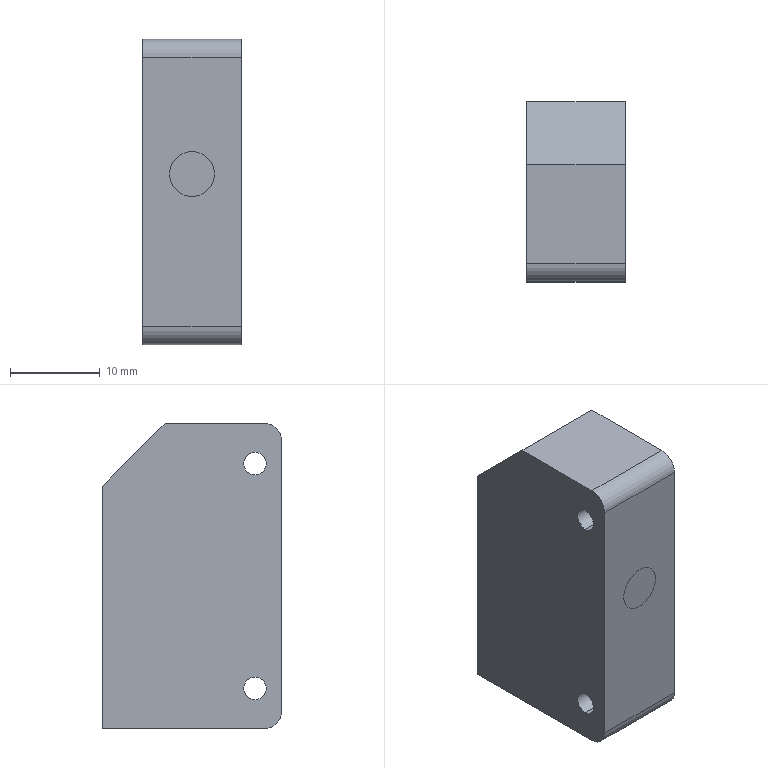Component | SolidWorks | MaterialDetectionSensor-1 | 1 solid | 14 faces | box 11 x 20 x 34 mm | volume 7084 mm3 | plane 8 | cylinder 6 | commonest cylinder face diameters 2.5 x4 4 x2
build123d program:
from build123d import *

# Parameters (mm, degrees)
SKETCH1_W           = 34
SKETCH1_H           = 20
BOSS_EXTRUDE1_DEPTH = 5.5
CUT_EXTRUDE1_DEPTH  = 23.583
M3_TAPPED_HOLE1_D   = 2.5
FILLET1_R           = 2


with BuildPart() as part:
    # Sketch1 → Boss-Extrude1 (new, symmetric)
    with BuildSketch(Plane.XY):
        Rectangle(SKETCH1_W, SKETCH1_H)
    extrude(amount=BOSS_EXTRUDE1_DEPTH, both=True)

    # Sketch2 → Cut-Extrude1 (cut, through all)
    with BuildSketch(Plane.XY.offset(5.5)):
        Polygon((-17, 10), (-10, 10), (-17, 3), align=None)
    extrude(amount=-CUT_EXTRUDE1_DEPTH, mode=Mode.SUBTRACT)

    # M3 Tapped Hole1 (through all)
    with Locations(Plane.XY.offset(5.5)):
        with Locations((-12.5, -7), (12.5, -7)):
            Hole(M3_TAPPED_HOLE1_D / 2)

    # Fillet1
    fillet1_edges = [part.edges().sort_by_distance(p)[0] for p in [
        (17, -10, 0),
        (-17, -10, 0),
    ]]
    fillet(fillet1_edges, radius=FILLET1_R)


solid = part.part

# Placed as in the assembly
solid = solid.moved(Location((-217.5, 1265.5, 90), (0, 90, 0)))
STEP:
#1=CARTESIAN_POINT('',(-8.78,49.547,4.085));
#2=VERTEX_POINT('',#1);
#3=CARTESIAN_POINT('',(-8.78,49.547,3.986));
#4=VERTEX_POINT('',#3);
#5=CARTESIAN_POINT('',(-8.78,49.547,4.035));
#6=DIRECTION('',(1.,0.,0.));
#7=DIRECTION('',(0.,0.,-1.));
#8=AXIS2_PLACEMENT_3D('',#5,#6,#7);
#9=CIRCLE('',#8,0.04921);
#10=EDGE_CURVE('',#2,#4,#9,.T.);
#11=ORIENTED_EDGE('',*,*,#10,.F.);
#12=CARTESIAN_POINT('',(-8.346,49.547,4.085));
#13=VERTEX_POINT('',#12);
#14=CARTESIAN_POINT('',(-8.346,49.547,4.085));
#15=DIRECTION('',(1.,0.,0.));
#16=VECTOR('',#15,39.37);
#17=LINE('',#14,#16);
#18=EDGE_CURVE('',#2,#13,#17,.T.);
#19=ORIENTED_EDGE('',*,*,#18,.T.);
#20=CARTESIAN_POINT('',(-8.346,49.547,3.986));
#21=VERTEX_POINT('',#20);
#22=CARTESIAN_POINT('',(-8.346,49.547,4.035));
#23=DIRECTION('',(1.,0.,0.));
#24=DIRECTION('',(0.,0.,-1.));
#25=AXIS2_PLACEMENT_3D('',#22,#23,#24);
#26=CIRCLE('',#25,0.04921);
#27=EDGE_CURVE('',#13,#21,#26,.T.);
#28=ORIENTED_EDGE('',*,*,#27,.T.);
#29=CARTESIAN_POINT('',(-8.346,49.547,3.986));
#30=DIRECTION('',(1.,0.,0.));
#31=VECTOR('',#30,39.37);
#32=LINE('',#29,#31);
#33=EDGE_CURVE('',#4,#21,#32,.T.);
#34=ORIENTED_EDGE('',*,*,#33,.F.);
#35=EDGE_LOOP('',(#11,#19,#28,#34));
#36=FACE_OUTER_BOUND('',#35,.T.);
#37=CARTESIAN_POINT('',(-8.346,49.547,4.035));
#38=DIRECTION('',(1.,0.,0.));
#39=DIRECTION('',(0.,0.,-1.));
#40=AXIS2_PLACEMENT_3D('',#37,#38,#39);
#41=CYLINDRICAL_SURFACE('',#40,0.04921);
#42=ADVANCED_FACE('',(#36),#41,.F.);
#43=CARTESIAN_POINT('',(-8.78,49.547,3.1));
#44=VERTEX_POINT('',#43);
#45=CARTESIAN_POINT('',(-8.78,49.547,3.002));
#46=VERTEX_POINT('',#45);
#47=CARTESIAN_POINT('',(-8.78,49.547,3.051));
#48=DIRECTION('',(1.,0.,0.));
#49=DIRECTION('',(0.,0.,-1.));
#50=AXIS2_PLACEMENT_3D('',#47,#48,#49);
#51=CIRCLE('',#50,0.04921);
#52=EDGE_CURVE('',#44,#46,#51,.T.);
#53=ORIENTED_EDGE('',*,*,#52,.F.);
#54=CARTESIAN_POINT('',(-8.346,49.547,3.1));
#55=VERTEX_POINT('',#54);
#56=CARTESIAN_POINT('',(-8.346,49.547,3.1));
#57=DIRECTION('',(1.,0.,0.));
#58=VECTOR('',#57,39.37);
#59=LINE('',#56,#58);
#60=EDGE_CURVE('',#44,#55,#59,.T.);
#61=ORIENTED_EDGE('',*,*,#60,.T.);
#62=CARTESIAN_POINT('',(-8.346,49.547,3.002));
#63=VERTEX_POINT('',#62);
#64=CARTESIAN_POINT('',(-8.346,49.547,3.051));
#65=DIRECTION('',(1.,0.,0.));
#66=DIRECTION('',(0.,0.,-1.));
#67=AXIS2_PLACEMENT_3D('',#64,#65,#66);
#68=CIRCLE('',#67,0.04921);
#69=EDGE_CURVE('',#55,#63,#68,.T.);
#70=ORIENTED_EDGE('',*,*,#69,.T.);
#71=CARTESIAN_POINT('',(-8.346,49.547,3.002));
#72=DIRECTION('',(1.,0.,0.));
#73=VECTOR('',#72,39.37);
#74=LINE('',#71,#73);
#75=EDGE_CURVE('',#46,#63,#74,.T.);
#76=ORIENTED_EDGE('',*,*,#75,.F.);
#77=EDGE_LOOP('',(#53,#61,#70,#76));
#78=FACE_OUTER_BOUND('',#77,.T.);
#79=CARTESIAN_POINT('',(-8.346,49.547,3.051));
#80=DIRECTION('',(1.,0.,0.));
#81=DIRECTION('',(0.,0.,-1.));
#82=AXIS2_PLACEMENT_3D('',#79,#80,#81);
#83=CYLINDRICAL_SURFACE('',#82,0.04921);
#84=ADVANCED_FACE('',(#78),#83,.F.);
#85=CARTESIAN_POINT('',(-8.346,49.429,4.134));
#86=VERTEX_POINT('',#85);
#87=CARTESIAN_POINT('',(-8.346,49.429,2.953));
#88=VERTEX_POINT('',#87);
#89=CARTESIAN_POINT('',(-8.346,49.429,4.213));
#90=DIRECTION('',(0.,-0.,-1.));
#91=VECTOR('',#90,39.37);
#92=LINE('',#89,#91);
#93=EDGE_CURVE('',#86,#88,#92,.T.);
#94=ORIENTED_EDGE('',*,*,#93,.F.);
#95=CARTESIAN_POINT('',(-8.78,49.429,4.134));
#96=VERTEX_POINT('',#95);
#97=CARTESIAN_POINT('',(-8.346,49.429,4.134));
#98=DIRECTION('',(-1.,-0.,0.));
#99=VECTOR('',#98,39.37);
#100=LINE('',#97,#99);
#101=EDGE_CURVE('',#86,#96,#100,.T.);
#102=ORIENTED_EDGE('',*,*,#101,.T.);
#103=CARTESIAN_POINT('',(-8.78,49.429,2.953));
#104=VERTEX_POINT('',#103);
#105=CARTESIAN_POINT('',(-8.78,49.429,4.213));
#106=DIRECTION('',(0.,-0.,-1.));
#107=VECTOR('',#106,39.37);
#108=LINE('',#105,#107);
#109=EDGE_CURVE('',#96,#104,#108,.T.);
#110=ORIENTED_EDGE('',*,*,#109,.T.);
#111=CARTESIAN_POINT('',(-8.346,49.429,2.953));
#112=DIRECTION('',(1.,0.,0.));
#113=VECTOR('',#112,39.37);
#114=LINE('',#111,#113);
#115=EDGE_CURVE('',#104,#88,#114,.T.);
#116=ORIENTED_EDGE('',*,*,#115,.T.);
#117=EDGE_LOOP('',(#94,#102,#110,#116));
#118=FACE_OUTER_BOUND('',#117,.T.);
#119=CARTESIAN_POINT('',(-8.465,49.429,3.622));
#120=VERTEX_POINT('',#119);
#121=CARTESIAN_POINT('',(-8.661,49.429,3.622));
#122=VERTEX_POINT('',#121);
#123=CARTESIAN_POINT('',(-8.563,49.429,3.622));
#124=DIRECTION('',(0.,-1.,0.));
#125=DIRECTION('',(1.,0.,0.));
#126=AXIS2_PLACEMENT_3D('',#123,#124,#125);
#127=CIRCLE('',#126,0.09843);
#128=EDGE_CURVE('',#120,#122,#127,.T.);
#129=ORIENTED_EDGE('',*,*,#128,.F.);
#130=CARTESIAN_POINT('',(-8.563,49.429,3.622));
#131=DIRECTION('',(0.,-1.,0.));
#132=DIRECTION('',(1.,0.,0.));
#133=AXIS2_PLACEMENT_3D('',#130,#131,#132);
#134=CIRCLE('',#133,0.09843);
#135=EDGE_CURVE('',#122,#120,#134,.T.);
#136=ORIENTED_EDGE('',*,*,#135,.F.);
#137=EDGE_LOOP('',(#129,#136));
#138=FACE_BOUND('',#137,.T.);
#139=CARTESIAN_POINT('',(-8.346,49.429,4.213));
#140=DIRECTION('',(-0.,1.,-0.));
#141=DIRECTION('',(1.,0.,0.));
#142=AXIS2_PLACEMENT_3D('',#139,#140,#141);
#143=PLANE('',#142);
#144=ADVANCED_FACE('',(#118,#138),#143,.F.);
#145=CARTESIAN_POINT('',(-8.346,49.508,2.874));
#146=VERTEX_POINT('',#145);
#147=CARTESIAN_POINT('',(-8.346,50.217,2.874));
#148=VERTEX_POINT('',#147);
#149=CARTESIAN_POINT('',(-8.346,50.217,2.874));
#150=DIRECTION('',(-0.,1.,-0.));
#151=VECTOR('',#150,39.37);
#152=LINE('',#149,#151);
#153=EDGE_CURVE('',#146,#148,#152,.T.);
#154=ORIENTED_EDGE('',*,*,#153,.F.);
#155=CARTESIAN_POINT('',(-8.78,49.508,2.874));
#156=VERTEX_POINT('',#155);
#157=CARTESIAN_POINT('',(-8.346,49.508,2.874));
#158=DIRECTION('',(-1.,-0.,0.));
#159=VECTOR('',#158,39.37);
#160=LINE('',#157,#159);
#161=EDGE_CURVE('',#146,#156,#160,.T.);
#162=ORIENTED_EDGE('',*,*,#161,.T.);
#163=CARTESIAN_POINT('',(-8.78,50.217,2.874));
#164=VERTEX_POINT('',#163);
#165=CARTESIAN_POINT('',(-8.78,50.217,2.874));
#166=DIRECTION('',(-0.,1.,-0.));
#167=VECTOR('',#166,39.37);
#168=LINE('',#165,#167);
#169=EDGE_CURVE('',#156,#164,#168,.T.);
#170=ORIENTED_EDGE('',*,*,#169,.T.);
#171=CARTESIAN_POINT('',(-8.346,50.217,2.874));
#172=DIRECTION('',(-1.,-0.,0.));
#173=VECTOR('',#172,39.37);
#174=LINE('',#171,#173);
#175=EDGE_CURVE('',#148,#164,#174,.T.);
#176=ORIENTED_EDGE('',*,*,#175,.F.);
#177=EDGE_LOOP('',(#154,#162,#170,#176));
#178=FACE_OUTER_BOUND('',#177,.T.);
#179=CARTESIAN_POINT('',(-8.346,50.217,2.874));
#180=DIRECTION('',(-0.,0.,1.));
#181=DIRECTION('',(1.,0.,0.));
#182=AXIS2_PLACEMENT_3D('',#179,#180,#181);
#183=PLANE('',#182);
#184=ADVANCED_FACE('',(#178),#183,.F.);
#185=CARTESIAN_POINT('',(-8.78,50.217,3.937));
#186=VERTEX_POINT('',#185);
#187=CARTESIAN_POINT('',(-8.78,50.217,4.213));
#188=DIRECTION('',(-0.,0.,1.));
#189=VECTOR('',#188,39.37);
#190=LINE('',#187,#189);
#191=EDGE_CURVE('',#164,#186,#190,.T.);
#192=ORIENTED_EDGE('',*,*,#191,.T.);
#193=CARTESIAN_POINT('',(-8.346,50.217,3.937));
#194=VERTEX_POINT('',#193);
#195=CARTESIAN_POINT('',(-8.78,50.217,3.937));
#196=DIRECTION('',(1.,0.,0.));
#197=VECTOR('',#196,39.37);
#198=LINE('',#195,#197);
#199=EDGE_CURVE('',#186,#194,#198,.T.);
#200=ORIENTED_EDGE('',*,*,#199,.T.);
#201=CARTESIAN_POINT('',(-8.346,50.217,4.213));
#202=DIRECTION('',(-0.,0.,1.));
#203=VECTOR('',#202,39.37);
#204=LINE('',#201,#203);
#205=EDGE_CURVE('',#148,#194,#204,.T.);
#206=ORIENTED_EDGE('',*,*,#205,.F.);
#207=ORIENTED_EDGE('',*,*,#175,.T.);
#208=EDGE_LOOP('',(#192,#200,#206,#207));
#209=FACE_OUTER_BOUND('',#208,.T.);
#210=CARTESIAN_POINT('',(-8.346,50.217,4.213));
#211=DIRECTION('',(0.,-1.,0.));
#212=DIRECTION('',(-1.,-0.,0.));
#213=AXIS2_PLACEMENT_3D('',#210,#211,#212);
#214=PLANE('',#213);
#215=ADVANCED_FACE('',(#209),#214,.F.);
#216=CARTESIAN_POINT('',(-8.78,49.941,4.213));
#217=VERTEX_POINT('',#216);
#218=CARTESIAN_POINT('',(-8.78,49.508,4.213));
#219=VERTEX_POINT('',#218);
#220=CARTESIAN_POINT('',(-8.78,50.217,4.213));
#221=DIRECTION('',(0.,-1.,0.));
#222=VECTOR('',#221,39.37);
#223=LINE('',#220,#222);
#224=EDGE_CURVE('',#217,#219,#223,.T.);
#225=ORIENTED_EDGE('',*,*,#224,.T.);
#226=CARTESIAN_POINT('',(-8.346,49.508,4.213));
#227=VERTEX_POINT('',#226);
#228=CARTESIAN_POINT('',(-8.346,49.508,4.213));
#229=DIRECTION('',(1.,0.,0.));
#230=VECTOR('',#229,39.37);
#231=LINE('',#228,#230);
#232=EDGE_CURVE('',#219,#227,#231,.T.);
#233=ORIENTED_EDGE('',*,*,#232,.T.);
#234=CARTESIAN_POINT('',(-8.346,49.941,4.213));
#235=VERTEX_POINT('',#234);
#236=CARTESIAN_POINT('',(-8.346,50.217,4.213));
#237=DIRECTION('',(0.,-1.,0.));
#238=VECTOR('',#237,39.37);
#239=LINE('',#236,#238);
#240=EDGE_CURVE('',#235,#227,#239,.T.);
#241=ORIENTED_EDGE('',*,*,#240,.F.);
#242=CARTESIAN_POINT('',(-8.78,49.941,4.213));
#243=DIRECTION('',(1.,0.,0.));
#244=VECTOR('',#243,39.37);
#245=LINE('',#242,#244);
#246=EDGE_CURVE('',#217,#235,#245,.T.);
#247=ORIENTED_EDGE('',*,*,#246,.F.);
#248=EDGE_LOOP('',(#225,#233,#241,#247));
#249=FACE_OUTER_BOUND('',#248,.T.);
#250=CARTESIAN_POINT('',(-8.346,50.217,4.213));
#251=DIRECTION('',(0.,-0.,-1.));
#252=DIRECTION('',(-1.,-0.,0.));
#253=AXIS2_PLACEMENT_3D('',#250,#251,#252);
#254=PLANE('',#253);
#255=ADVANCED_FACE('',(#249),#254,.F.);
#256=ORIENTED_EDGE('',*,*,#128,.T.);
#257=ORIENTED_EDGE('',*,*,#135,.T.);
#258=EDGE_LOOP('',(#256,#257));
#259=FACE_OUTER_BOUND('',#258,.T.);
#260=CARTESIAN_POINT('',(-8.346,49.429,4.213));
#261=DIRECTION('',(-0.,1.,-0.));
#262=DIRECTION('',(1.,0.,0.));
#263=AXIS2_PLACEMENT_3D('',#260,#261,#262);
#264=PLANE('',#263);
#265=ADVANCED_FACE('',(#259),#264,.F.);
#266=CARTESIAN_POINT('',(-8.346,49.547,4.035));
#267=DIRECTION('',(1.,0.,0.));
#268=DIRECTION('',(0.,0.,-1.));
#269=AXIS2_PLACEMENT_3D('',#266,#267,#268);
#270=CIRCLE('',#269,0.04921);
#271=EDGE_CURVE('',#21,#13,#270,.T.);
#272=ORIENTED_EDGE('',*,*,#271,.F.);
#273=ORIENTED_EDGE('',*,*,#27,.F.);
#274=EDGE_LOOP('',(#272,#273));
#275=FACE_BOUND('',#274,.T.);
#276=CARTESIAN_POINT('',(-8.346,49.547,3.051));
#277=DIRECTION('',(1.,0.,0.));
#278=DIRECTION('',(0.,0.,-1.));
#279=AXIS2_PLACEMENT_3D('',#276,#277,#278);
#280=CIRCLE('',#279,0.04921);
#281=EDGE_CURVE('',#63,#55,#280,.T.);
#282=ORIENTED_EDGE('',*,*,#281,.F.);
#283=ORIENTED_EDGE('',*,*,#69,.F.);
#284=EDGE_LOOP('',(#282,#283));
#285=FACE_BOUND('',#284,.T.);
#286=ORIENTED_EDGE('',*,*,#240,.T.);
#287=CARTESIAN_POINT('',(-8.346,49.508,4.134));
#288=DIRECTION('',(1.,0.,0.));
#289=DIRECTION('',(0.,0.,-1.));
#290=AXIS2_PLACEMENT_3D('',#287,#288,#289);
#291=CIRCLE('',#290,0.07874);
#292=EDGE_CURVE('',#227,#86,#291,.T.);
#293=ORIENTED_EDGE('',*,*,#292,.T.);
#294=ORIENTED_EDGE('',*,*,#93,.T.);
#295=CARTESIAN_POINT('',(-8.346,49.508,2.953));
#296=DIRECTION('',(1.,0.,0.));
#297=DIRECTION('',(0.,0.,-1.));
#298=AXIS2_PLACEMENT_3D('',#295,#296,#297);
#299=CIRCLE('',#298,0.07874);
#300=EDGE_CURVE('',#88,#146,#299,.T.);
#301=ORIENTED_EDGE('',*,*,#300,.T.);
#302=ORIENTED_EDGE('',*,*,#153,.T.);
#303=ORIENTED_EDGE('',*,*,#205,.T.);
#304=CARTESIAN_POINT('',(-8.346,50.217,3.937));
#305=DIRECTION('',(-0.,0.7071,-0.7071));
#306=VECTOR('',#305,39.37);
#307=LINE('',#304,#306);
#308=EDGE_CURVE('',#235,#194,#307,.T.);
#309=ORIENTED_EDGE('',*,*,#308,.F.);
#310=EDGE_LOOP('',(#286,#293,#294,#301,#302,#303,#309));
#311=FACE_OUTER_BOUND('',#310,.T.);
#312=CARTESIAN_POINT('',(-8.346,49.823,3.543));
#313=DIRECTION('',(1.,0.,0.));
#314=DIRECTION('',(0.,-0.,-1.));
#315=AXIS2_PLACEMENT_3D('',#312,#313,#314);
#316=PLANE('',#315);
#317=ADVANCED_FACE('',(#275,#285,#311),#316,.T.);
#318=CARTESIAN_POINT('',(-8.78,49.547,4.035));
#319=DIRECTION('',(1.,0.,0.));
#320=DIRECTION('',(0.,0.,-1.));
#321=AXIS2_PLACEMENT_3D('',#318,#319,#320);
#322=CIRCLE('',#321,0.04921);
#323=EDGE_CURVE('',#4,#2,#322,.T.);
#324=ORIENTED_EDGE('',*,*,#323,.T.);
#325=ORIENTED_EDGE('',*,*,#10,.T.);
#326=EDGE_LOOP('',(#324,#325));
#327=FACE_BOUND('',#326,.T.);
#328=CARTESIAN_POINT('',(-8.78,49.547,3.051));
#329=DIRECTION('',(1.,0.,0.));
#330=DIRECTION('',(0.,0.,-1.));
#331=AXIS2_PLACEMENT_3D('',#328,#329,#330);
#332=CIRCLE('',#331,0.04921);
#333=EDGE_CURVE('',#46,#44,#332,.T.);
#334=ORIENTED_EDGE('',*,*,#333,.T.);
#335=ORIENTED_EDGE('',*,*,#52,.T.);
#336=EDGE_LOOP('',(#334,#335));
#337=FACE_BOUND('',#336,.T.);
#338=ORIENTED_EDGE('',*,*,#109,.F.);
#339=CARTESIAN_POINT('',(-8.78,49.508,4.134));
#340=DIRECTION('',(-1.,-0.,0.));
#341=DIRECTION('',(0.,0.,-1.));
#342=AXIS2_PLACEMENT_3D('',#339,#340,#341);
#343=CIRCLE('',#342,0.07874);
#344=EDGE_CURVE('',#96,#219,#343,.T.);
#345=ORIENTED_EDGE('',*,*,#344,.T.);
#346=ORIENTED_EDGE('',*,*,#224,.F.);
#347=CARTESIAN_POINT('',(-8.78,50.217,3.937));
#348=DIRECTION('',(-0.,0.7071,-0.7071));
#349=VECTOR('',#348,39.37);
#350=LINE('',#347,#349);
#351=EDGE_CURVE('',#217,#186,#350,.T.);
#352=ORIENTED_EDGE('',*,*,#351,.T.);
#353=ORIENTED_EDGE('',*,*,#191,.F.);
#354=ORIENTED_EDGE('',*,*,#169,.F.);
#355=CARTESIAN_POINT('',(-8.78,49.508,2.953));
#356=DIRECTION('',(-1.,-0.,0.));
#357=DIRECTION('',(0.,0.,-1.));
#358=AXIS2_PLACEMENT_3D('',#355,#356,#357);
#359=CIRCLE('',#358,0.07874);
#360=EDGE_CURVE('',#156,#104,#359,.T.);
#361=ORIENTED_EDGE('',*,*,#360,.T.);
#362=EDGE_LOOP('',(#338,#345,#346,#352,#353,#354,#361));
#363=FACE_OUTER_BOUND('',#362,.T.);
#364=CARTESIAN_POINT('',(-8.78,49.823,3.543));
#365=DIRECTION('',(1.,0.,0.));
#366=DIRECTION('',(0.,-0.,-1.));
#367=AXIS2_PLACEMENT_3D('',#364,#365,#366);
#368=PLANE('',#367);
#369=ADVANCED_FACE('',(#327,#337,#363),#368,.F.);
#370=ORIENTED_EDGE('',*,*,#308,.T.);
#371=ORIENTED_EDGE('',*,*,#199,.F.);
#372=ORIENTED_EDGE('',*,*,#351,.F.);
#373=ORIENTED_EDGE('',*,*,#246,.T.);
#374=EDGE_LOOP('',(#370,#371,#372,#373));
#375=FACE_OUTER_BOUND('',#374,.T.);
#376=CARTESIAN_POINT('',(-8.78,50.217,3.937));
#377=DIRECTION('',(0.,-0.7071,-0.7071));
#378=DIRECTION('',(-0.,0.7071,-0.7071));
#379=AXIS2_PLACEMENT_3D('',#376,#377,#378);
#380=PLANE('',#379);
#381=ADVANCED_FACE('',(#375),#380,.F.);
#382=ORIENTED_EDGE('',*,*,#60,.F.);
#383=ORIENTED_EDGE('',*,*,#333,.F.);
#384=ORIENTED_EDGE('',*,*,#75,.T.);
#385=ORIENTED_EDGE('',*,*,#281,.T.);
#386=EDGE_LOOP('',(#382,#383,#384,#385));
#387=FACE_OUTER_BOUND('',#386,.T.);
#388=CARTESIAN_POINT('',(-8.346,49.547,3.051));
#389=DIRECTION('',(1.,0.,0.));
#390=DIRECTION('',(0.,0.,-1.));
#391=AXIS2_PLACEMENT_3D('',#388,#389,#390);
#392=CYLINDRICAL_SURFACE('',#391,0.04921);
#393=ADVANCED_FACE('',(#387),#392,.F.);
#394=ORIENTED_EDGE('',*,*,#18,.F.);
#395=ORIENTED_EDGE('',*,*,#323,.F.);
#396=ORIENTED_EDGE('',*,*,#33,.T.);
#397=ORIENTED_EDGE('',*,*,#271,.T.);
#398=EDGE_LOOP('',(#394,#395,#396,#397));
#399=FACE_OUTER_BOUND('',#398,.T.);
#400=CARTESIAN_POINT('',(-8.346,49.547,4.035));
#401=DIRECTION('',(1.,0.,0.));
#402=DIRECTION('',(0.,0.,-1.));
#403=AXIS2_PLACEMENT_3D('',#400,#401,#402);
#404=CYLINDRICAL_SURFACE('',#403,0.04921);
#405=ADVANCED_FACE('',(#399),#404,.F.);
#406=ORIENTED_EDGE('',*,*,#292,.F.);
#407=ORIENTED_EDGE('',*,*,#232,.F.);
#408=ORIENTED_EDGE('',*,*,#344,.F.);
#409=ORIENTED_EDGE('',*,*,#101,.F.);
#410=EDGE_LOOP('',(#406,#407,#408,#409));
#411=FACE_OUTER_BOUND('',#410,.T.);
#412=CARTESIAN_POINT('',(-8.346,49.508,4.134));
#413=DIRECTION('',(-1.,-0.,0.));
#414=DIRECTION('',(0.,0.,1.));
#415=AXIS2_PLACEMENT_3D('',#412,#413,#414);
#416=CYLINDRICAL_SURFACE('',#415,0.07874);
#417=ADVANCED_FACE('',(#411),#416,.T.);
#418=ORIENTED_EDGE('',*,*,#300,.F.);
#419=ORIENTED_EDGE('',*,*,#115,.F.);
#420=ORIENTED_EDGE('',*,*,#360,.F.);
#421=ORIENTED_EDGE('',*,*,#161,.F.);
#422=EDGE_LOOP('',(#418,#419,#420,#421));
#423=FACE_OUTER_BOUND('',#422,.T.);
#424=CARTESIAN_POINT('',(-8.346,49.508,2.953));
#425=DIRECTION('',(-1.,-0.,0.));
#426=DIRECTION('',(0.,0.,1.));
#427=AXIS2_PLACEMENT_3D('',#424,#425,#426);
#428=CYLINDRICAL_SURFACE('',#427,0.07874);
#429=ADVANCED_FACE('',(#423),#428,.T.);
#430=CLOSED_SHELL('',(#42,#84,#144,#184,#215,#255,#265,#317,#369,#381,#393,#405,#417,#429));
#431=MANIFOLD_SOLID_BREP('',#430);
#432=CARTESIAN_POINT('',(0.,0.,0.));
#433=DIRECTION('',(0.,0.,1.));
#434=DIRECTION('',(1.,0.,0.));
#435=AXIS2_PLACEMENT_3D('',#432,#433,#434);
#436=(LENGTH_UNIT()NAMED_UNIT(*)SI_UNIT($,.METRE.));
#437=LENGTH_MEASURE_WITH_UNIT(LENGTH_MEASURE(0.0254),#436);
#438=DIMENSIONAL_EXPONENTS(1.,0.,0.,0.,0.,0.,0.);
#439=(CONVERSION_BASED_UNIT('',#437)LENGTH_UNIT()NAMED_UNIT(#438));
#440=UNCERTAINTY_MEASURE_WITH_UNIT(LENGTH_MEASURE(0.00001),#439,'','');
#441=(NAMED_UNIT(*)PLANE_ANGLE_UNIT()SI_UNIT($,.RADIAN.));
#442=(NAMED_UNIT(*)SI_UNIT($,.STERADIAN.)SOLID_ANGLE_UNIT());
#443=(GEOMETRIC_REPRESENTATION_CONTEXT(3)GLOBAL_UNCERTAINTY_ASSIGNED_CONTEXT((#440))GLOBAL_UNIT_ASSIGNED_CONTEXT((#439,#441,#442))REPRESENTATION_CONTEXT('',''));
#444=ADVANCED_BREP_SHAPE_REPRESENTATION('',(#431,#435),#443);
#445=COLOUR_RGB('',0.7922,0.8196,0.9333);
#446=FILL_AREA_STYLE_COLOUR('',#445);
#447=FILL_AREA_STYLE('',(#446));
#448=SURFACE_STYLE_FILL_AREA(#447);
#449=SURFACE_SIDE_STYLE('',(#448));
#450=SURFACE_STYLE_USAGE(.BOTH.,#449);
#451=PRESENTATION_STYLE_ASSIGNMENT((#450));
#452=STYLED_ITEM('',(#451),#431);
#453=PRESENTATION_LAYER_ASSIGNMENT('','',(#452));
#454=(LENGTH_UNIT()NAMED_UNIT(*)SI_UNIT($,.METRE.));
#455=LENGTH_MEASURE_WITH_UNIT(LENGTH_MEASURE(0.0254),#454);
#456=DIMENSIONAL_EXPONENTS(1.,0.,0.,0.,0.,0.,0.);
#457=(CONVERSION_BASED_UNIT('',#455)LENGTH_UNIT()NAMED_UNIT(#456));
#458=UNCERTAINTY_MEASURE_WITH_UNIT(LENGTH_MEASURE(0.00001),#457,'','');
#459=(NAMED_UNIT(*)PLANE_ANGLE_UNIT()SI_UNIT($,.RADIAN.));
#460=(NAMED_UNIT(*)SI_UNIT($,.STERADIAN.)SOLID_ANGLE_UNIT());
#461=(GEOMETRIC_REPRESENTATION_CONTEXT(3)GLOBAL_UNCERTAINTY_ASSIGNED_CONTEXT((#458))GLOBAL_UNIT_ASSIGNED_CONTEXT((#457,#459,#460))REPRESENTATION_CONTEXT('',''));
#462=MECHANICAL_DESIGN_GEOMETRIC_PRESENTATION_REPRESENTATION('',(#452),#461);